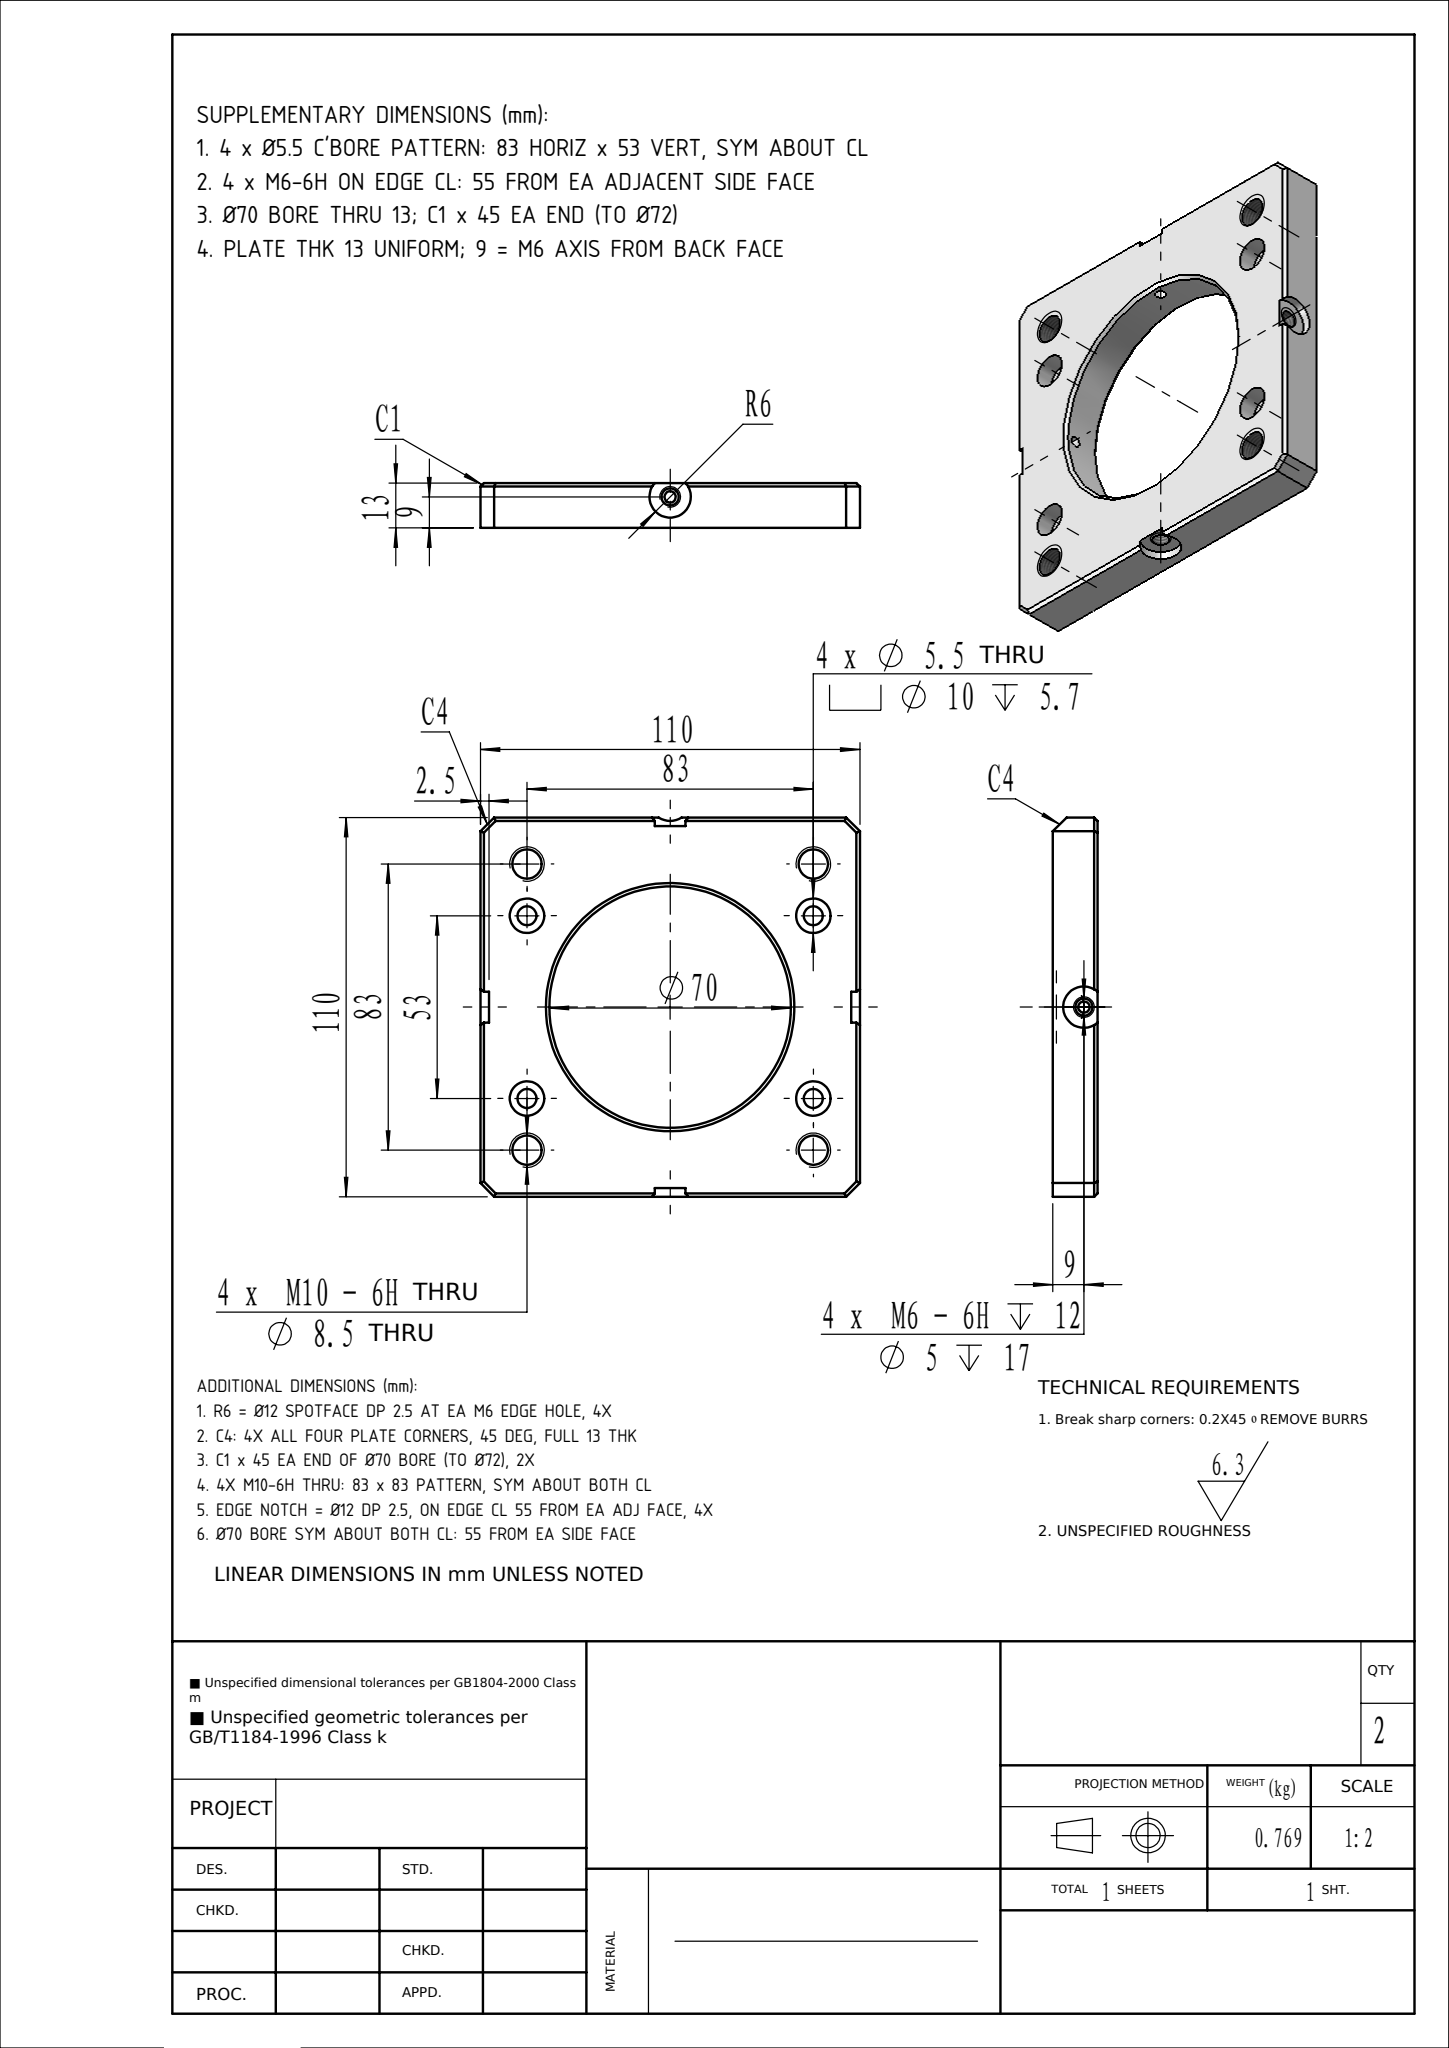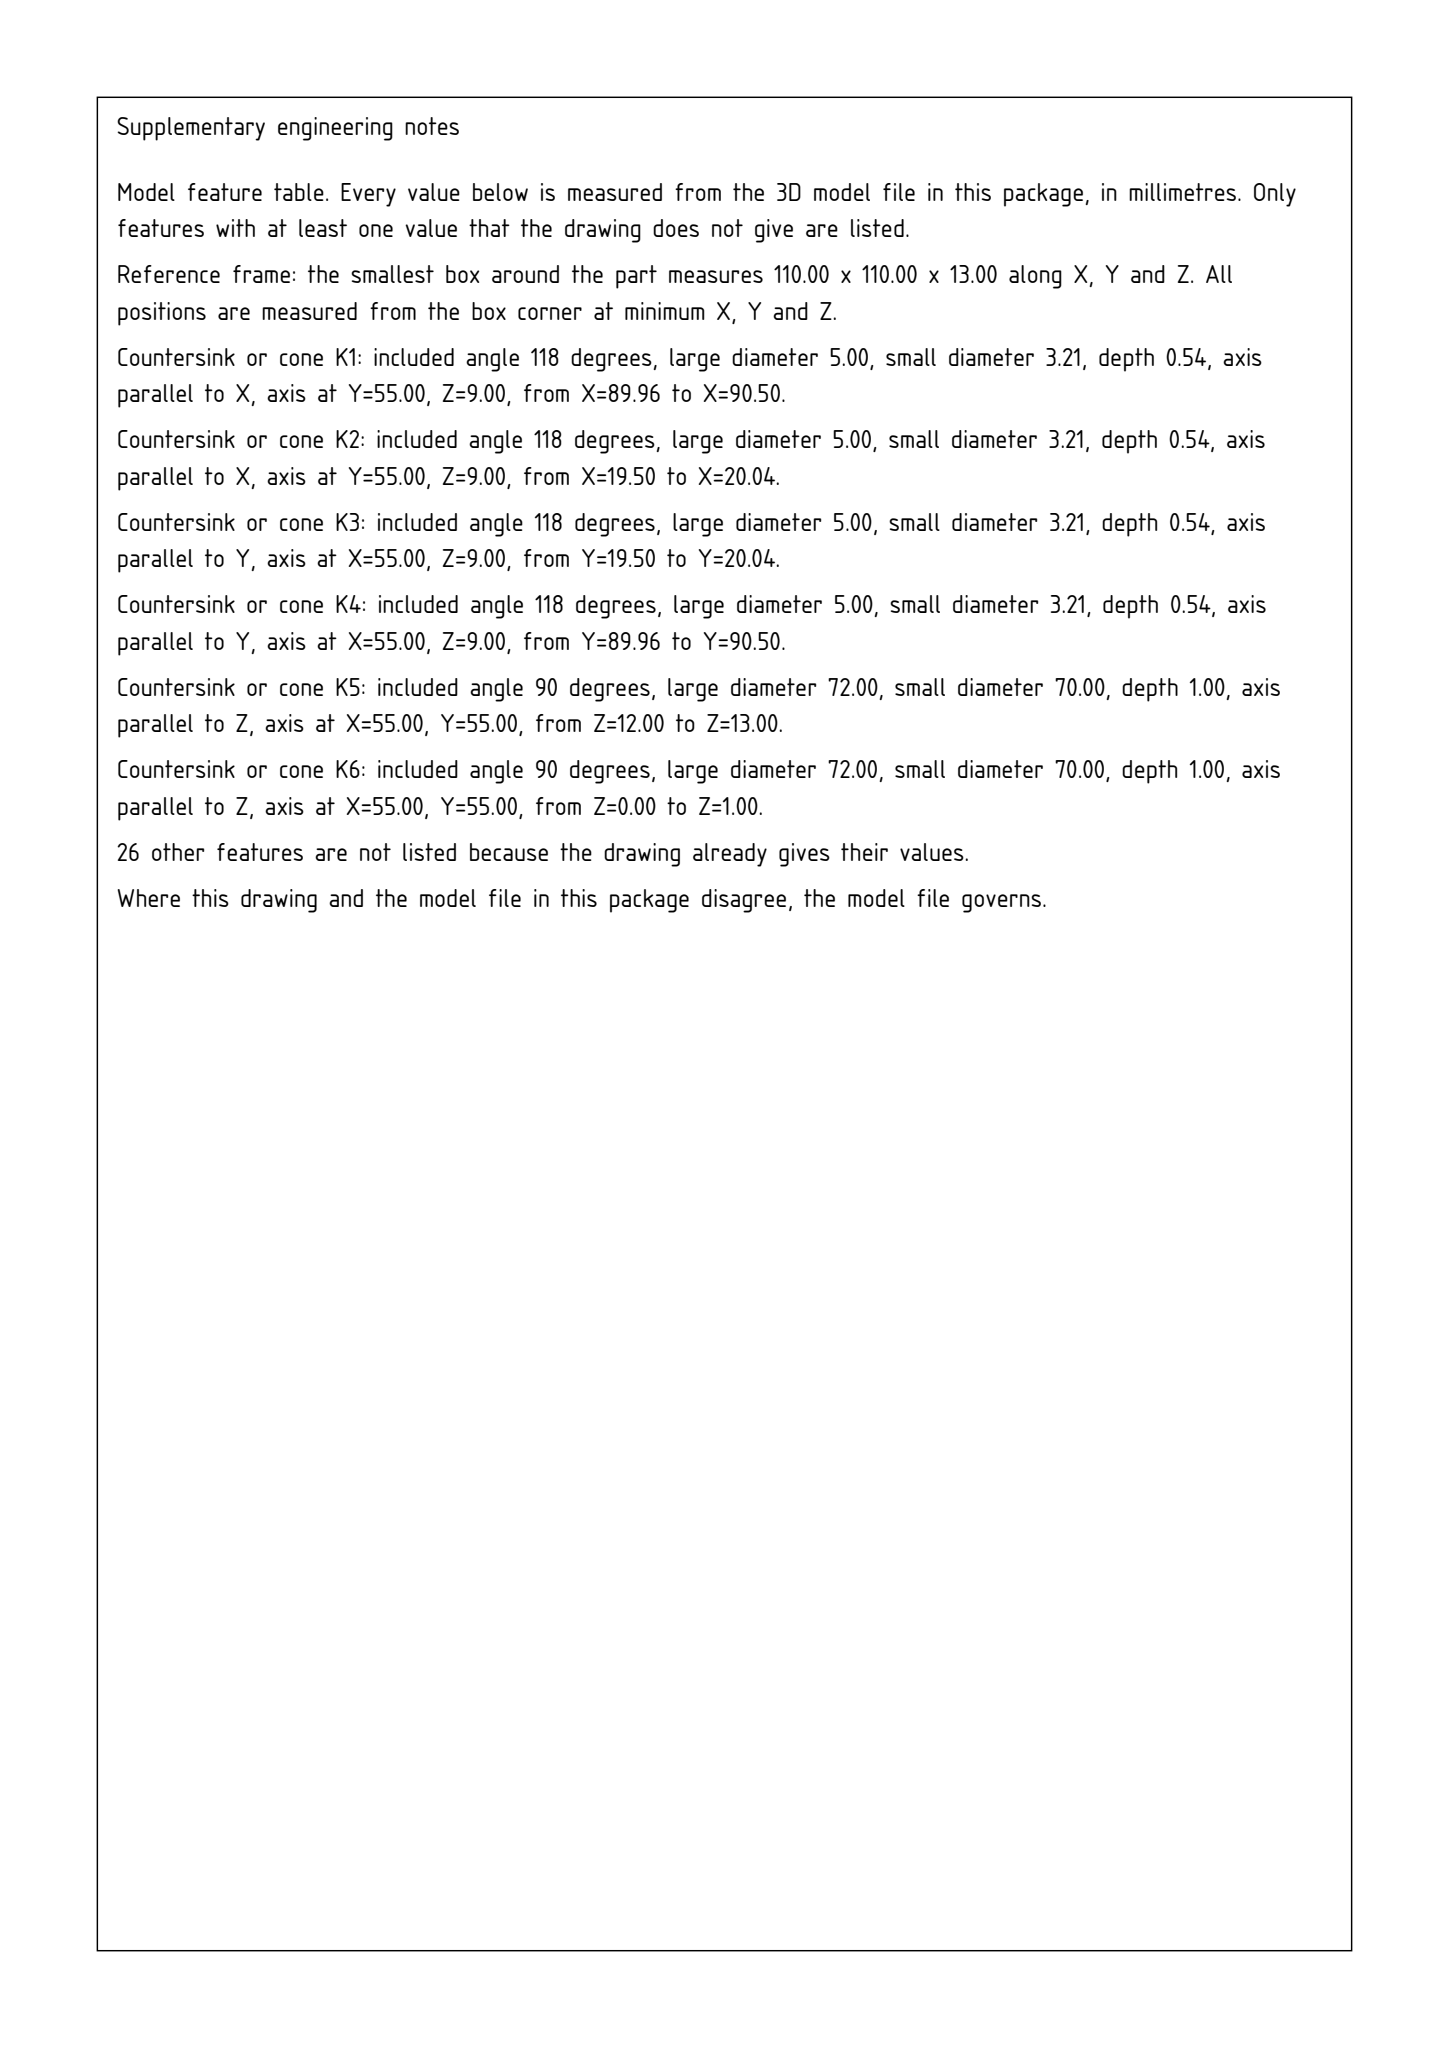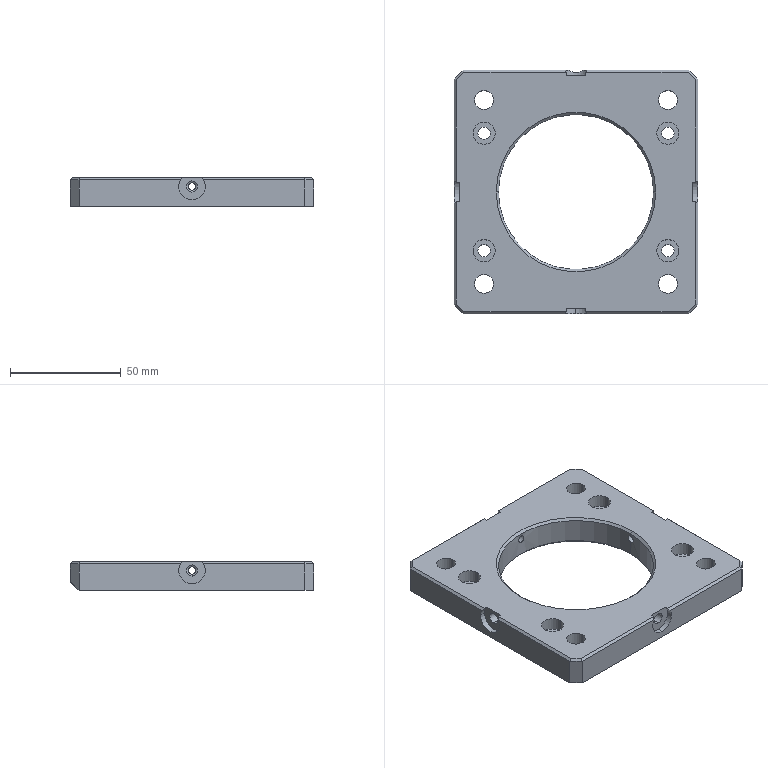Part | SolidWorks | mm | 1 solid | 87 faces | box 110 x 110 x 13 mm | volume 97796 mm3 | cylinder 43 | plane 32 | cone 12 | commonest cylinder face diameters 12 x9 10 x8 5.5 x8 5 x8 8.5 x8 70 x2